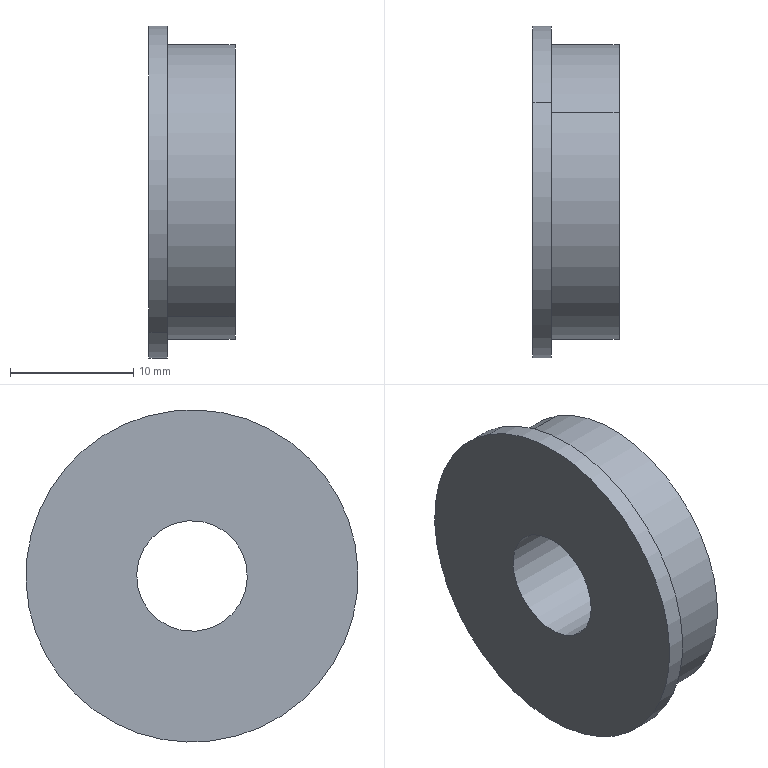Component | SolidWorks | F609ZZ(Battery)122-1 | 1 solid | 9 faces | box 7 x 27 x 27 mm | volume 2902 mm3 | cylinder 6 | plane 3 | commonest cylinder face diameters 9 x2 27 x2 24 x2
build123d program:
from build123d import *


with BuildPart() as part:
    # Sketch2 → Revolve1 (revolve)
    with BuildSketch(Plane.XY, mode=Mode.PRIVATE) as revolve1_sk:
        Polygon((12, 7), (12, 1.5), (13.5, 1.5), (13.5, 0), (4.5, 0), (4.5, 7), align=None)
    revolve(revolve1_sk.sketch.rotate(Axis((0, 0, 0), (0, 1, 0)), 90), axis=Axis((0, 0, 0), (0, 1, 0)))


solid = part.part

# Placed as in the assembly
solid = solid.moved(Location((-231.979, 448.741, 848.5), (0, 0, -90)))
STEP:
#1=COLOUR_RGB('',0.7922,0.8196,0.9333);
#2=FILL_AREA_STYLE_COLOUR('',#1);
#3=FILL_AREA_STYLE('',(#2));
#4=SURFACE_STYLE_FILL_AREA(#3);
#5=SURFACE_SIDE_STYLE('',(#4));
#6=SURFACE_STYLE_USAGE(.BOTH.,#5);
#7=PRESENTATION_STYLE_ASSIGNMENT((#6));
#8=CARTESIAN_POINT('',(-8.857,17.762,33.555));
#9=VERTEX_POINT('',#8);
#10=CARTESIAN_POINT('',(-8.857,17.572,33.256));
#11=VERTEX_POINT('',#10);
#12=CARTESIAN_POINT('',(-8.857,17.667,33.406));
#13=DIRECTION('',(-1.,0.,0.));
#14=DIRECTION('',(0.,-0.5364,-0.844));
#15=AXIS2_PLACEMENT_3D('',#12,#13,#14);
#16=CIRCLE('',#15,0.1772);
#17=EDGE_CURVE('',#9,#11,#16,.T.);
#18=ORIENTED_EDGE('',*,*,#17,.F.);
#19=CARTESIAN_POINT('',(-9.133,17.762,33.555));
#20=VERTEX_POINT('',#19);
#21=CARTESIAN_POINT('',(-9.133,17.762,33.555));
#22=DIRECTION('',(-1.,0.,0.));
#23=VECTOR('',#22,39.37);
#24=LINE('',#21,#23);
#25=EDGE_CURVE('',#9,#20,#24,.T.);
#26=ORIENTED_EDGE('',*,*,#25,.T.);
#27=CARTESIAN_POINT('',(-9.133,17.572,33.256));
#28=VERTEX_POINT('',#27);
#29=CARTESIAN_POINT('',(-9.133,17.667,33.406));
#30=DIRECTION('',(-1.,0.,0.));
#31=DIRECTION('',(0.,-0.5364,-0.844));
#32=AXIS2_PLACEMENT_3D('',#29,#30,#31);
#33=CIRCLE('',#32,0.1772);
#34=EDGE_CURVE('',#20,#28,#33,.T.);
#35=ORIENTED_EDGE('',*,*,#34,.T.);
#36=CARTESIAN_POINT('',(-9.133,17.572,33.256));
#37=DIRECTION('',(-1.,0.,0.));
#38=VECTOR('',#37,39.37);
#39=LINE('',#36,#38);
#40=EDGE_CURVE('',#11,#28,#39,.T.);
#41=ORIENTED_EDGE('',*,*,#40,.F.);
#42=EDGE_LOOP('',(#18,#26,#35,#41));
#43=FACE_OUTER_BOUND('',#42,.T.);
#44=CARTESIAN_POINT('',(-9.133,17.667,33.406));
#45=DIRECTION('',(-1.,0.,0.));
#46=DIRECTION('',(0.,-0.5364,-0.844));
#47=AXIS2_PLACEMENT_3D('',#44,#45,#46);
#48=CYLINDRICAL_SURFACE('',#47,0.1772);
#49=ADVANCED_FACE('',(#43),#48,.F.);
#50=CARTESIAN_POINT('',(-9.074,17.382,32.957));
#51=VERTEX_POINT('',#50);
#52=CARTESIAN_POINT('',(-9.074,17.952,33.854));
#53=VERTEX_POINT('',#52);
#54=CARTESIAN_POINT('',(-9.074,17.667,33.406));
#55=DIRECTION('',(-1.,0.,0.));
#56=DIRECTION('',(0.,-0.5364,-0.844));
#57=AXIS2_PLACEMENT_3D('',#54,#55,#56);
#58=CIRCLE('',#57,0.5315);
#59=EDGE_CURVE('',#51,#53,#58,.T.);
#60=ORIENTED_EDGE('',*,*,#59,.T.);
#61=CARTESIAN_POINT('',(-9.133,17.952,33.854));
#62=VERTEX_POINT('',#61);
#63=CARTESIAN_POINT('',(-9.133,17.952,33.854));
#64=DIRECTION('',(-1.,0.,0.));
#65=VECTOR('',#64,39.37);
#66=LINE('',#63,#65);
#67=EDGE_CURVE('',#53,#62,#66,.T.);
#68=ORIENTED_EDGE('',*,*,#67,.T.);
#69=CARTESIAN_POINT('',(-9.133,17.382,32.957));
#70=VERTEX_POINT('',#69);
#71=CARTESIAN_POINT('',(-9.133,17.667,33.406));
#72=DIRECTION('',(-1.,0.,0.));
#73=DIRECTION('',(0.,-0.5364,-0.844));
#74=AXIS2_PLACEMENT_3D('',#71,#72,#73);
#75=CIRCLE('',#74,0.5315);
#76=EDGE_CURVE('',#70,#62,#75,.T.);
#77=ORIENTED_EDGE('',*,*,#76,.F.);
#78=CARTESIAN_POINT('',(-9.133,17.382,32.957));
#79=DIRECTION('',(-1.,0.,0.));
#80=VECTOR('',#79,39.37);
#81=LINE('',#78,#80);
#82=EDGE_CURVE('',#51,#70,#81,.T.);
#83=ORIENTED_EDGE('',*,*,#82,.F.);
#84=EDGE_LOOP('',(#60,#68,#77,#83));
#85=FACE_OUTER_BOUND('',#84,.T.);
#86=CARTESIAN_POINT('',(-9.133,17.667,33.406));
#87=DIRECTION('',(-1.,0.,0.));
#88=DIRECTION('',(0.,-0.5364,-0.844));
#89=AXIS2_PLACEMENT_3D('',#86,#87,#88);
#90=CYLINDRICAL_SURFACE('',#89,0.5315);
#91=ADVANCED_FACE('',(#85),#90,.T.);
#92=CARTESIAN_POINT('',(-8.857,17.414,33.007));
#93=VERTEX_POINT('',#92);
#94=CARTESIAN_POINT('',(-8.857,17.92,33.804));
#95=VERTEX_POINT('',#94);
#96=CARTESIAN_POINT('',(-8.857,17.667,33.406));
#97=DIRECTION('',(-1.,0.,0.));
#98=DIRECTION('',(0.,-0.5364,-0.844));
#99=AXIS2_PLACEMENT_3D('',#96,#97,#98);
#100=CIRCLE('',#99,0.4724);
#101=EDGE_CURVE('',#93,#95,#100,.T.);
#102=ORIENTED_EDGE('',*,*,#101,.T.);
#103=CARTESIAN_POINT('',(-9.074,17.92,33.804));
#104=VERTEX_POINT('',#103);
#105=CARTESIAN_POINT('',(-9.133,17.92,33.804));
#106=DIRECTION('',(-1.,0.,0.));
#107=VECTOR('',#106,39.37);
#108=LINE('',#105,#107);
#109=EDGE_CURVE('',#95,#104,#108,.T.);
#110=ORIENTED_EDGE('',*,*,#109,.T.);
#111=CARTESIAN_POINT('',(-9.074,17.414,33.007));
#112=VERTEX_POINT('',#111);
#113=CARTESIAN_POINT('',(-9.074,17.667,33.406));
#114=DIRECTION('',(-1.,0.,0.));
#115=DIRECTION('',(0.,-0.5364,-0.844));
#116=AXIS2_PLACEMENT_3D('',#113,#114,#115);
#117=CIRCLE('',#116,0.4724);
#118=EDGE_CURVE('',#112,#104,#117,.T.);
#119=ORIENTED_EDGE('',*,*,#118,.F.);
#120=CARTESIAN_POINT('',(-9.133,17.414,33.007));
#121=DIRECTION('',(-1.,0.,0.));
#122=VECTOR('',#121,39.37);
#123=LINE('',#120,#122);
#124=EDGE_CURVE('',#93,#112,#123,.T.);
#125=ORIENTED_EDGE('',*,*,#124,.F.);
#126=EDGE_LOOP('',(#102,#110,#119,#125));
#127=FACE_OUTER_BOUND('',#126,.T.);
#128=CARTESIAN_POINT('',(-9.133,17.667,33.406));
#129=DIRECTION('',(-1.,0.,0.));
#130=DIRECTION('',(0.,-0.5364,-0.844));
#131=AXIS2_PLACEMENT_3D('',#128,#129,#130);
#132=CYLINDRICAL_SURFACE('',#131,0.4724);
#133=ADVANCED_FACE('',(#127),#132,.T.);
#134=CARTESIAN_POINT('',(-8.857,17.667,33.406));
#135=DIRECTION('',(-1.,0.,0.));
#136=DIRECTION('',(0.,-0.5364,-0.844));
#137=AXIS2_PLACEMENT_3D('',#134,#135,#136);
#138=CIRCLE('',#137,0.1772);
#139=EDGE_CURVE('',#11,#9,#138,.T.);
#140=ORIENTED_EDGE('',*,*,#139,.T.);
#141=ORIENTED_EDGE('',*,*,#17,.T.);
#142=EDGE_LOOP('',(#140,#141));
#143=FACE_BOUND('',#142,.T.);
#144=ORIENTED_EDGE('',*,*,#101,.F.);
#145=CARTESIAN_POINT('',(-8.857,17.667,33.406));
#146=DIRECTION('',(-1.,0.,0.));
#147=DIRECTION('',(0.,-0.5364,-0.844));
#148=AXIS2_PLACEMENT_3D('',#145,#146,#147);
#149=CIRCLE('',#148,0.4724);
#150=EDGE_CURVE('',#95,#93,#149,.T.);
#151=ORIENTED_EDGE('',*,*,#150,.F.);
#152=EDGE_LOOP('',(#144,#151));
#153=FACE_OUTER_BOUND('',#152,.T.);
#154=CARTESIAN_POINT('',(-8.857,17.517,33.501));
#155=DIRECTION('',(1.,0.,0.));
#156=DIRECTION('',(0.,0.5364,0.844));
#157=AXIS2_PLACEMENT_3D('',#154,#155,#156);
#158=PLANE('',#157);
#159=ADVANCED_FACE('',(#143,#153),#158,.T.);
#160=ORIENTED_EDGE('',*,*,#109,.F.);
#161=ORIENTED_EDGE('',*,*,#150,.T.);
#162=ORIENTED_EDGE('',*,*,#124,.T.);
#163=CARTESIAN_POINT('',(-9.074,17.667,33.406));
#164=DIRECTION('',(-1.,0.,0.));
#165=DIRECTION('',(0.,-0.5364,-0.844));
#166=AXIS2_PLACEMENT_3D('',#163,#164,#165);
#167=CIRCLE('',#166,0.4724);
#168=EDGE_CURVE('',#104,#112,#167,.T.);
#169=ORIENTED_EDGE('',*,*,#168,.F.);
#170=EDGE_LOOP('',(#160,#161,#162,#169));
#171=FACE_OUTER_BOUND('',#170,.T.);
#172=CARTESIAN_POINT('',(-9.133,17.667,33.406));
#173=DIRECTION('',(-1.,0.,0.));
#174=DIRECTION('',(0.,-0.5364,-0.844));
#175=AXIS2_PLACEMENT_3D('',#172,#173,#174);
#176=CYLINDRICAL_SURFACE('',#175,0.4724);
#177=ADVANCED_FACE('',(#171),#176,.T.);
#178=ORIENTED_EDGE('',*,*,#118,.T.);
#179=ORIENTED_EDGE('',*,*,#168,.T.);
#180=EDGE_LOOP('',(#178,#179));
#181=FACE_BOUND('',#180,.T.);
#182=ORIENTED_EDGE('',*,*,#59,.F.);
#183=CARTESIAN_POINT('',(-9.074,17.667,33.406));
#184=DIRECTION('',(-1.,0.,0.));
#185=DIRECTION('',(0.,-0.5364,-0.844));
#186=AXIS2_PLACEMENT_3D('',#183,#184,#185);
#187=CIRCLE('',#186,0.5315);
#188=EDGE_CURVE('',#53,#51,#187,.T.);
#189=ORIENTED_EDGE('',*,*,#188,.F.);
#190=EDGE_LOOP('',(#182,#189));
#191=FACE_OUTER_BOUND('',#190,.T.);
#192=CARTESIAN_POINT('',(-9.074,17.268,33.659));
#193=DIRECTION('',(1.,0.,0.));
#194=DIRECTION('',(0.,0.5364,0.844));
#195=AXIS2_PLACEMENT_3D('',#192,#193,#194);
#196=PLANE('',#195);
#197=ADVANCED_FACE('',(#181,#191),#196,.T.);
#198=ORIENTED_EDGE('',*,*,#67,.F.);
#199=ORIENTED_EDGE('',*,*,#188,.T.);
#200=ORIENTED_EDGE('',*,*,#82,.T.);
#201=CARTESIAN_POINT('',(-9.133,17.667,33.406));
#202=DIRECTION('',(-1.,0.,0.));
#203=DIRECTION('',(0.,-0.5364,-0.844));
#204=AXIS2_PLACEMENT_3D('',#201,#202,#203);
#205=CIRCLE('',#204,0.5315);
#206=EDGE_CURVE('',#62,#70,#205,.T.);
#207=ORIENTED_EDGE('',*,*,#206,.F.);
#208=EDGE_LOOP('',(#198,#199,#200,#207));
#209=FACE_OUTER_BOUND('',#208,.T.);
#210=CARTESIAN_POINT('',(-9.133,17.667,33.406));
#211=DIRECTION('',(-1.,0.,0.));
#212=DIRECTION('',(0.,-0.5364,-0.844));
#213=AXIS2_PLACEMENT_3D('',#210,#211,#212);
#214=CYLINDRICAL_SURFACE('',#213,0.5315);
#215=ADVANCED_FACE('',(#209),#214,.T.);
#216=ORIENTED_EDGE('',*,*,#76,.T.);
#217=ORIENTED_EDGE('',*,*,#206,.T.);
#218=EDGE_LOOP('',(#216,#217));
#219=FACE_OUTER_BOUND('',#218,.T.);
#220=CARTESIAN_POINT('',(-9.133,17.667,33.406));
#221=DIRECTION('',(-1.,0.,0.));
#222=DIRECTION('',(0.,-0.5364,-0.844));
#223=AXIS2_PLACEMENT_3D('',#220,#221,#222);
#224=CIRCLE('',#223,0.1772);
#225=EDGE_CURVE('',#28,#20,#224,.T.);
#226=ORIENTED_EDGE('',*,*,#225,.F.);
#227=ORIENTED_EDGE('',*,*,#34,.F.);
#228=EDGE_LOOP('',(#226,#227));
#229=FACE_BOUND('',#228,.T.);
#230=CARTESIAN_POINT('',(-9.133,17.218,33.691));
#231=DIRECTION('',(-1.,0.,0.));
#232=DIRECTION('',(0.,-0.5364,-0.844));
#233=AXIS2_PLACEMENT_3D('',#230,#231,#232);
#234=PLANE('',#233);
#235=ADVANCED_FACE('',(#219,#229),#234,.T.);
#236=ORIENTED_EDGE('',*,*,#25,.F.);
#237=ORIENTED_EDGE('',*,*,#139,.F.);
#238=ORIENTED_EDGE('',*,*,#40,.T.);
#239=ORIENTED_EDGE('',*,*,#225,.T.);
#240=EDGE_LOOP('',(#236,#237,#238,#239));
#241=FACE_OUTER_BOUND('',#240,.T.);
#242=CARTESIAN_POINT('',(-9.133,17.667,33.406));
#243=DIRECTION('',(-1.,0.,0.));
#244=DIRECTION('',(0.,-0.5364,-0.844));
#245=AXIS2_PLACEMENT_3D('',#242,#243,#244);
#246=CYLINDRICAL_SURFACE('',#245,0.1772);
#247=ADVANCED_FACE('',(#241),#246,.F.);
#248=CLOSED_SHELL('',(#49,#91,#133,#159,#177,#197,#215,#235,#247));
#249=MANIFOLD_SOLID_BREP('',#248);
#250=STYLED_ITEM('',(#7),#249);
#251=(LENGTH_UNIT()NAMED_UNIT(*)SI_UNIT($,.METRE.));
#252=LENGTH_MEASURE_WITH_UNIT(LENGTH_MEASURE(0.0254),#251);
#253=DIMENSIONAL_EXPONENTS(1.,0.,0.,0.,0.,0.,0.);
#254=(CONVERSION_BASED_UNIT('',#252)LENGTH_UNIT()NAMED_UNIT(#253));
#255=UNCERTAINTY_MEASURE_WITH_UNIT(LENGTH_MEASURE(0.00001),#254,'','');
#256=(NAMED_UNIT(*)PLANE_ANGLE_UNIT()SI_UNIT($,.RADIAN.));
#257=(NAMED_UNIT(*)SI_UNIT($,.STERADIAN.)SOLID_ANGLE_UNIT());
#258=(GEOMETRIC_REPRESENTATION_CONTEXT(3)GLOBAL_UNCERTAINTY_ASSIGNED_CONTEXT((#255))GLOBAL_UNIT_ASSIGNED_CONTEXT((#254,#256,#257))REPRESENTATION_CONTEXT('',''));
#259=MECHANICAL_DESIGN_GEOMETRIC_PRESENTATION_REPRESENTATION('',(#250),#258);
#260=CARTESIAN_POINT('',(0.,0.,0.));
#261=DIRECTION('',(0.,0.,1.));
#262=DIRECTION('',(1.,0.,0.));
#263=AXIS2_PLACEMENT_3D('',#260,#261,#262);
#264=(LENGTH_UNIT()NAMED_UNIT(*)SI_UNIT($,.METRE.));
#265=LENGTH_MEASURE_WITH_UNIT(LENGTH_MEASURE(0.0254),#264);
#266=DIMENSIONAL_EXPONENTS(1.,0.,0.,0.,0.,0.,0.);
#267=(CONVERSION_BASED_UNIT('',#265)LENGTH_UNIT()NAMED_UNIT(#266));
#268=UNCERTAINTY_MEASURE_WITH_UNIT(LENGTH_MEASURE(0.00001),#267,'','');
#269=(NAMED_UNIT(*)PLANE_ANGLE_UNIT()SI_UNIT($,.RADIAN.));
#270=(NAMED_UNIT(*)SI_UNIT($,.STERADIAN.)SOLID_ANGLE_UNIT());
#271=(GEOMETRIC_REPRESENTATION_CONTEXT(3)GLOBAL_UNCERTAINTY_ASSIGNED_CONTEXT((#268))GLOBAL_UNIT_ASSIGNED_CONTEXT((#267,#269,#270))REPRESENTATION_CONTEXT('',''));
#272=ADVANCED_BREP_SHAPE_REPRESENTATION('',(#249,#263),#271);
#273=PRESENTATION_LAYER_ASSIGNMENT('','',(#250));